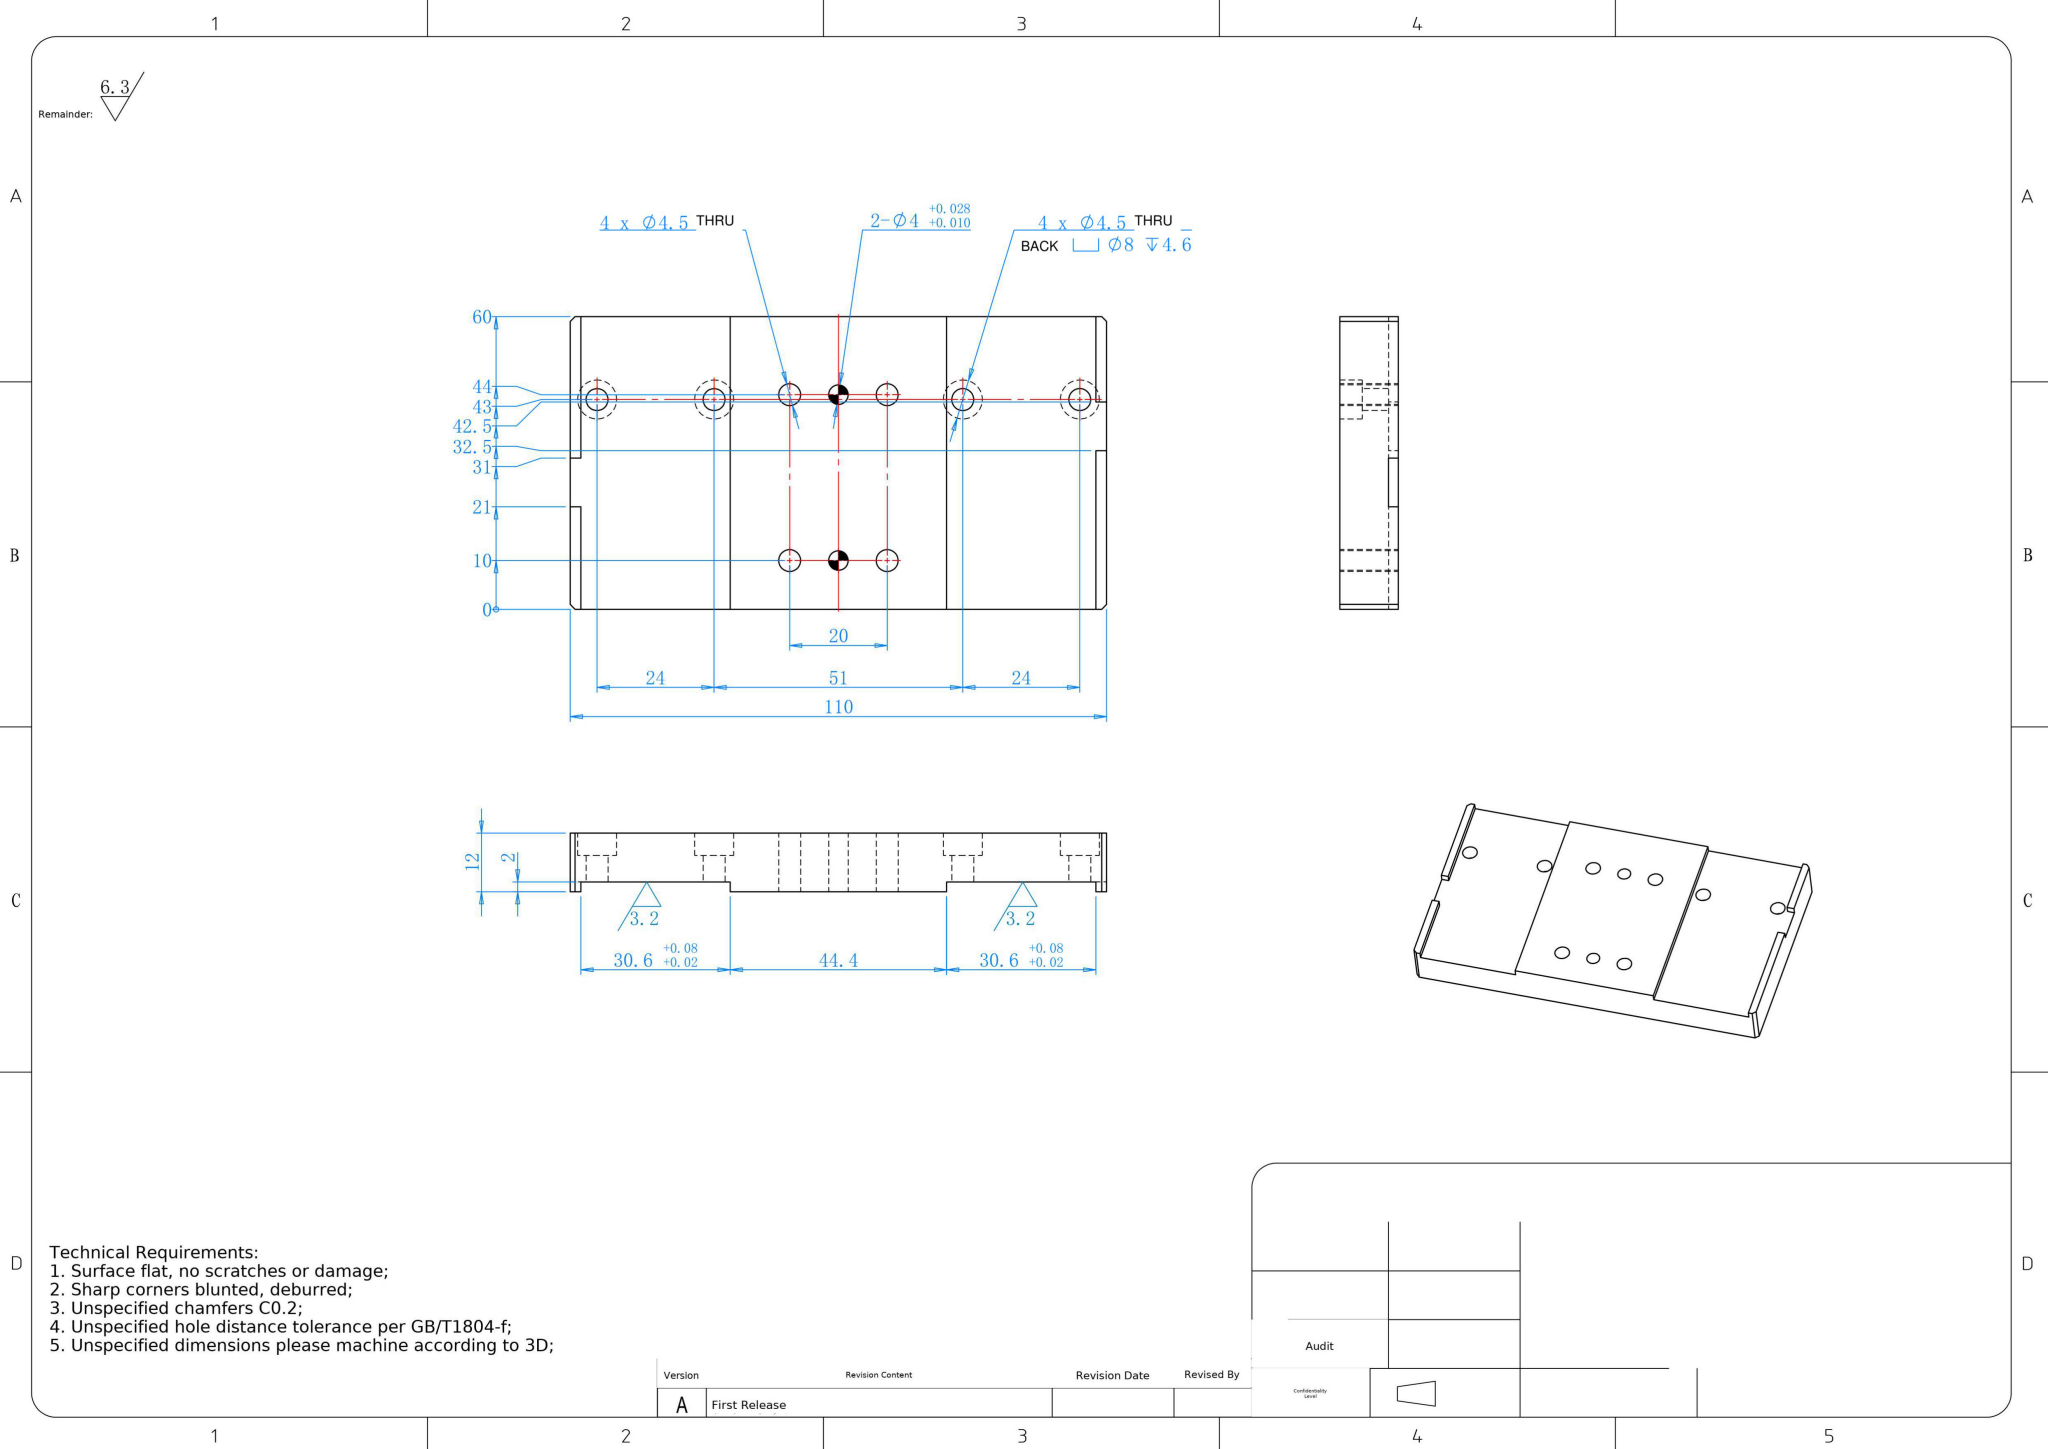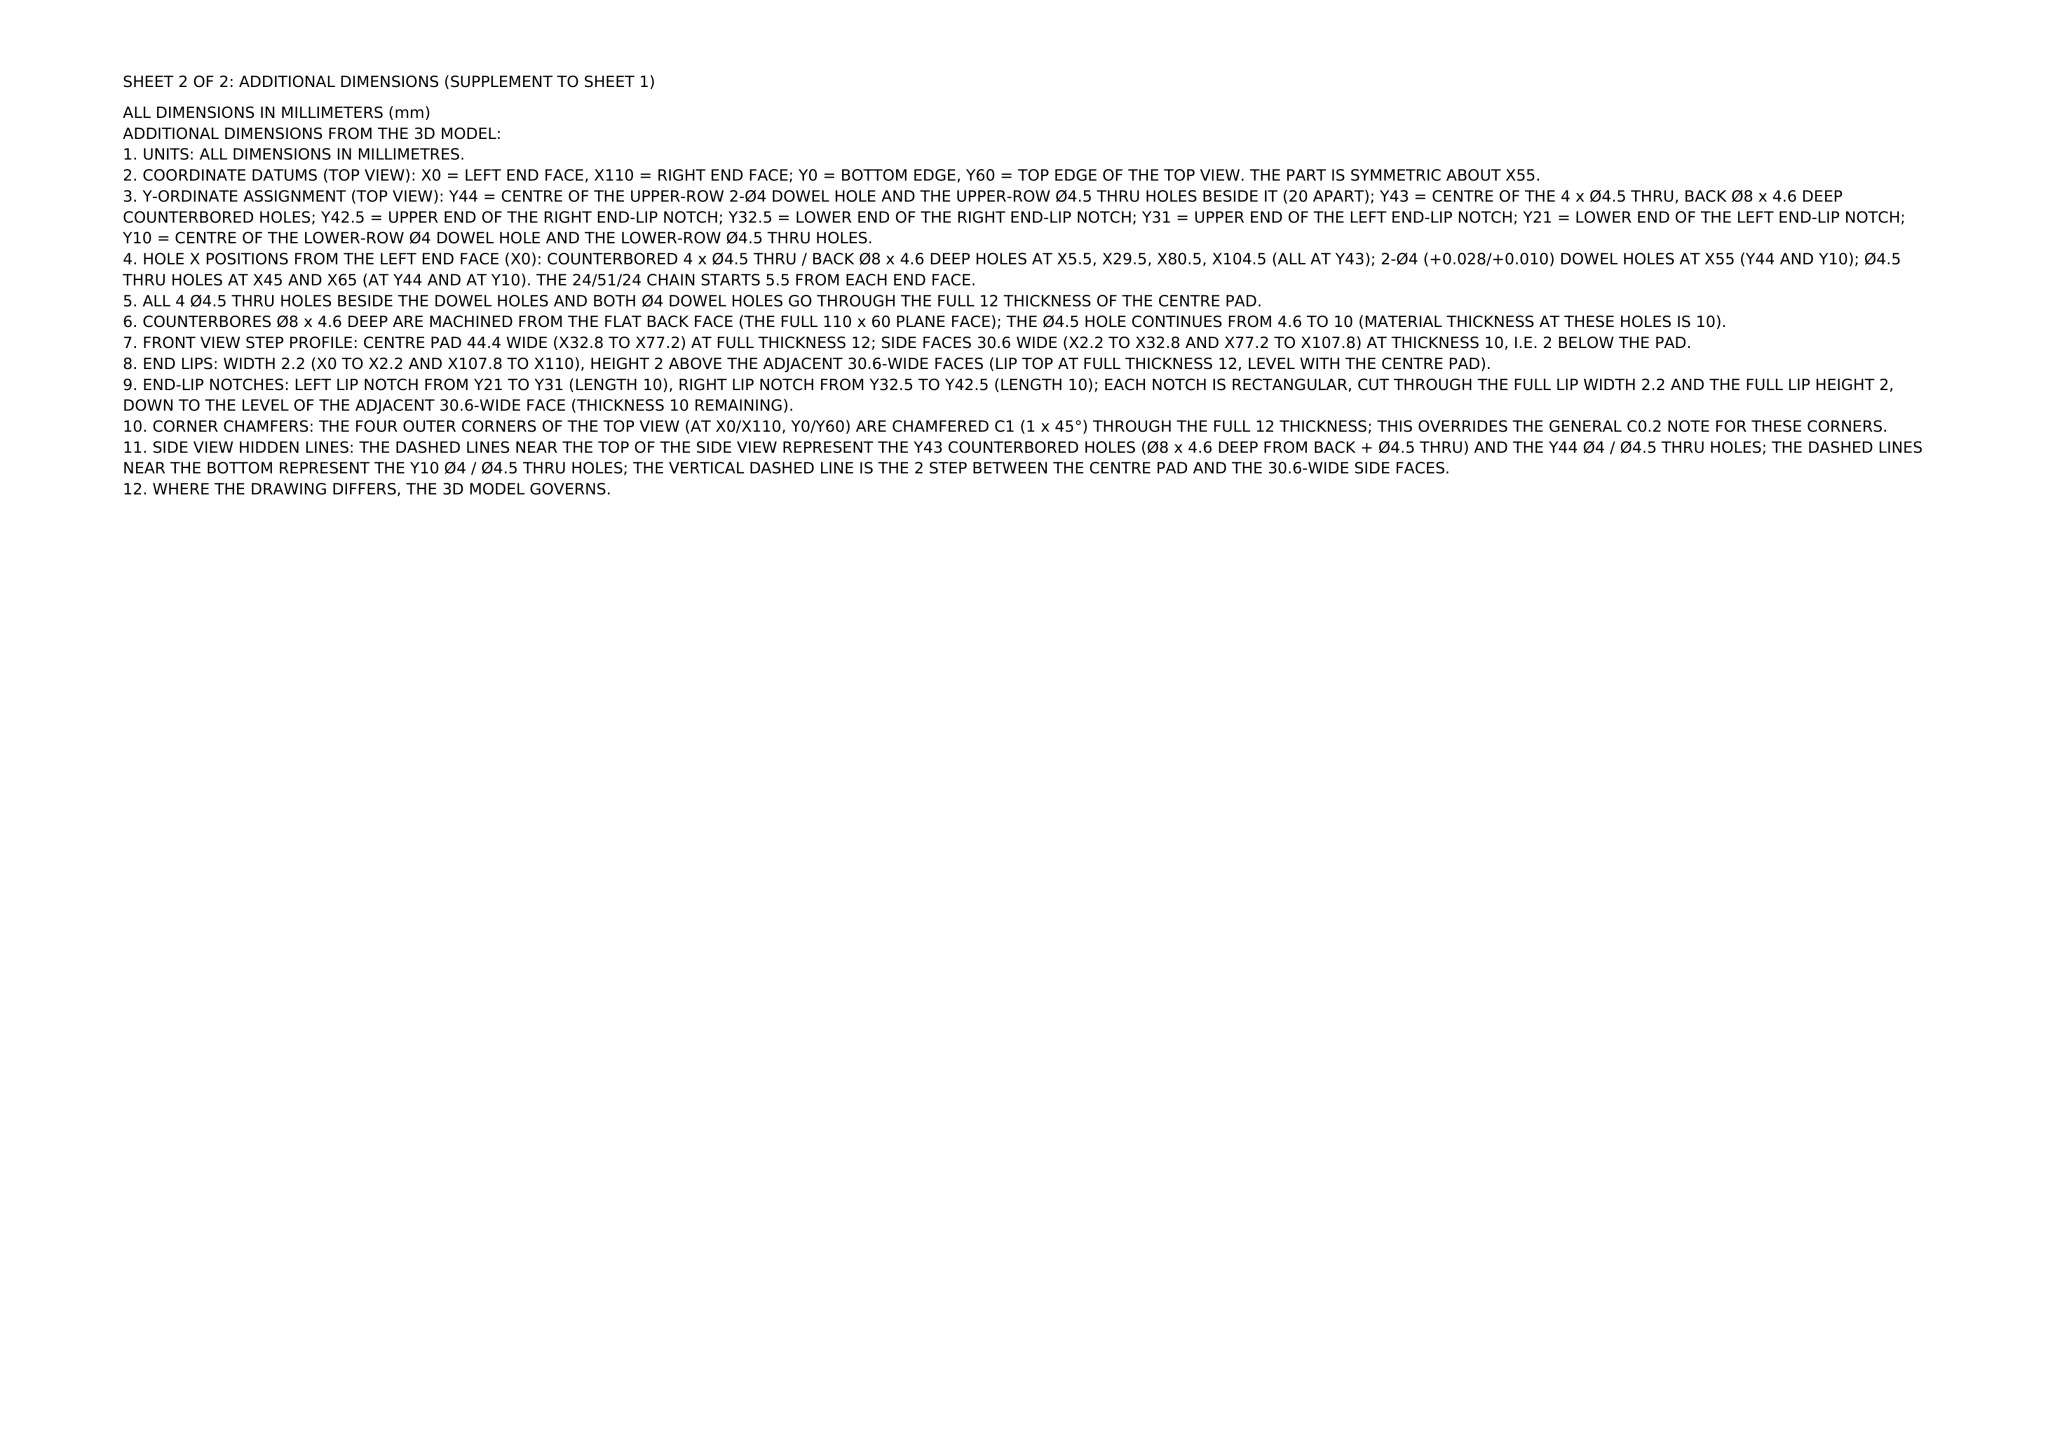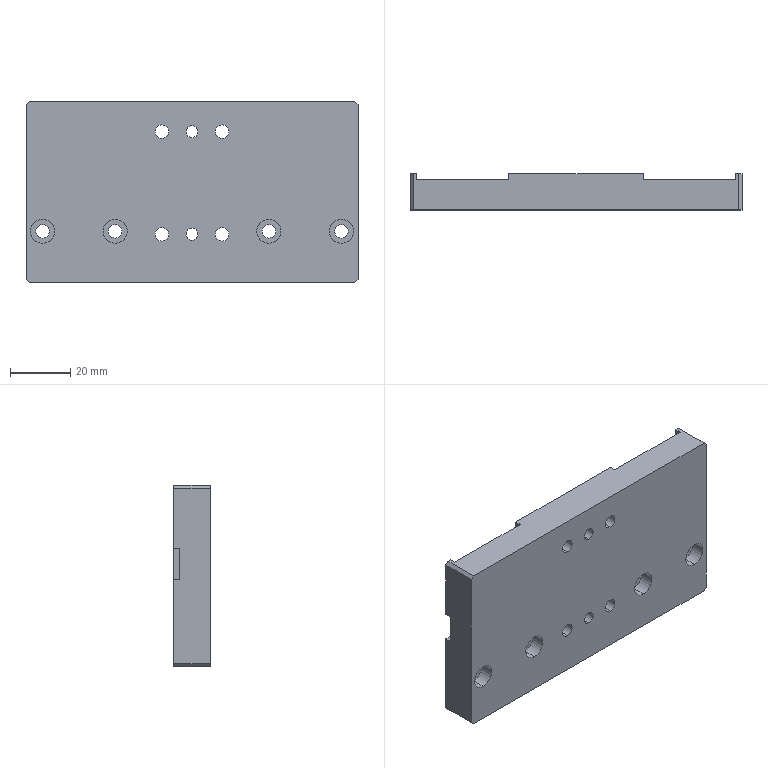Part | NX | mm | Stepped Edge Dual-Tab Rectangular Mounting Bracket | 1 solid | 58 faces | box 110 x 12 x 60 mm | volume 69411 mm3 | plane 30 | cylinder 28 | commonest cylinder face diameters 4.5 x16 8 x8 4 x4